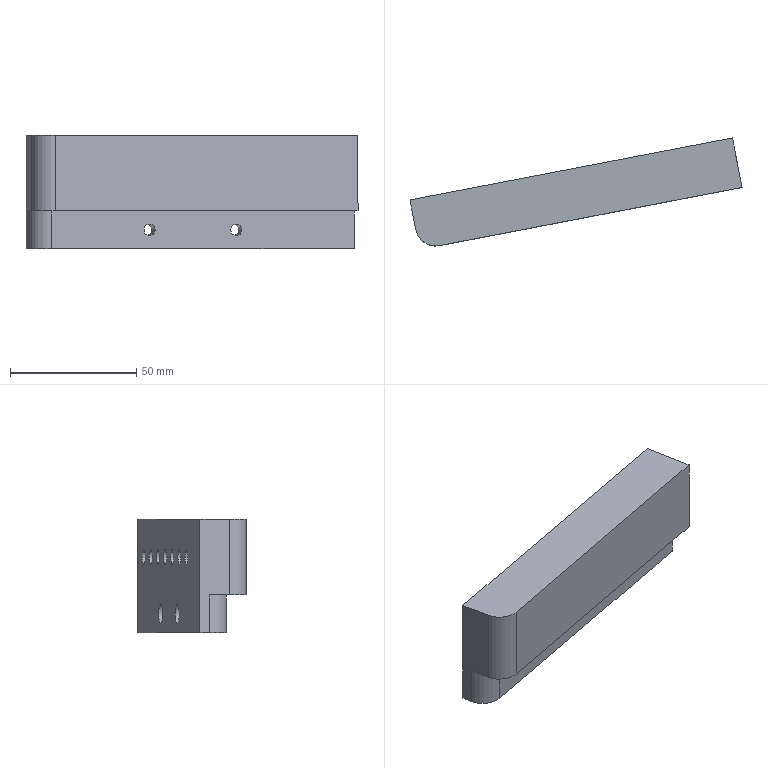Component | SolidWorks | SuctionCupMountingBlock2-1 | 1 solid | 37 faces | box 131.44 x 42.78 x 45 mm | volume 90210 mm3 | cylinder 26 | plane 11 | commonest cylinder face diameters 6 x14 8 x4 4.5 x4 10 x2 16 x2
build123d program:
from build123d import *

# Parameters (mm, degrees)
SKETCH2_W                                       = 20
SKETCH2_H                                       = 130
BOSS_EXTRUDE1_DEPTH                             = 30
SKETCH3_W                                       = 15
SKETCH3_H                                       = 130
BOSS_EXTRUDE2_DEPTH                             = 12
SKETCH4_R                                       = 3
CUT_EXTRUDE1_DEPTH                              = 11
SKETCH5_R                                       = 5
CUT_EXTRUDE2_DEPTH                              = 110
M4_HEX_SOCKET_HEAD_CAP_SCREW_CBORE1_D           = 4.5
M4_HEX_SOCKET_HEAD_CAP_SCREW_CBORE1_DEPTH       = 20
M4_HEX_SOCKET_HEAD_CAP_SCREW_CBORE1_CBORE_D     = 8
M4_HEX_SOCKET_HEAD_CAP_SCREW_CBORE1_CBORE_DEPTH = 4.6
M4_HEX_SOCKET_HEAD_CAP_SCREW_CBORE1_TIP         = 1.352
FILLET1_R                                       = 8


with BuildPart() as part:
    # Sketch2 → Boss-Extrude1 (new body)
    with BuildSketch(Plane.XY):
        with Locations((10, 65)):
            Rectangle(SKETCH2_W, SKETCH2_H)
    extrude(amount=BOSS_EXTRUDE1_DEPTH)

    # Sketch3 → Boss-Extrude2 (add)
    with BuildSketch(Plane(origin=(20, 0, 0), x_dir=(0, 0, -1), z_dir=(1, 0, 0))):
        with Locations((-37.5, 65)):
            Rectangle(SKETCH3_W, SKETCH3_H)
    extrude(amount=-BOSS_EXTRUDE2_DEPTH)

    # Sketch4 → Cut-Extrude1 (cut)
    with BuildSketch(Plane(origin=(20, 0, 0), x_dir=(0, 0, -1), z_dir=(1, 0, 0))):
        with Locations((-15, 118)):
            Circle(SKETCH4_R)
        with Locations((-15, 103)):
            Circle(SKETCH4_R)
        with Locations((-15, 88)):
            Circle(SKETCH4_R)
        with Locations((-15, 73)):
            Circle(SKETCH4_R)
        with Locations((-15, 58)):
            Circle(SKETCH4_R)
        with Locations((-15, 43)):
            Circle(SKETCH4_R)
        with Locations((-15, 28)):
            Circle(SKETCH4_R)
    extrude(amount=-CUT_EXTRUDE1_DEPTH, mode=Mode.SUBTRACT)

    # Sketch5 → Cut-Extrude2 (cut)
    with BuildSketch(Plane(origin=(0, 130, 0), x_dir=(1, 0, 0), z_dir=(0, 1, 0))):
        with Locations(Location((9, -15, 0), (0, 0, 270))):
            Circle(SKETCH5_R)
    extrude(amount=-CUT_EXTRUDE2_DEPTH, mode=Mode.SUBTRACT)

    # M4 Hex Socket Head Cap Screw CBORE1
    with Locations(Plane(origin=(20, 0, 0), x_dir=(0, 0, -1), z_dir=(1, 0, 0))):
        with Locations((-37.5, 82.5), (-37.5, 47.5)):
            CounterBoreHole(M4_HEX_SOCKET_HEAD_CAP_SCREW_CBORE1_D / 2, M4_HEX_SOCKET_HEAD_CAP_SCREW_CBORE1_CBORE_D / 2, M4_HEX_SOCKET_HEAD_CAP_SCREW_CBORE1_CBORE_DEPTH, depth=M4_HEX_SOCKET_HEAD_CAP_SCREW_CBORE1_DEPTH)
            with Locations((0, 0, -(M4_HEX_SOCKET_HEAD_CAP_SCREW_CBORE1_DEPTH + M4_HEX_SOCKET_HEAD_CAP_SCREW_CBORE1_TIP / 2))):  # 118° drill point
                Cone(0, M4_HEX_SOCKET_HEAD_CAP_SCREW_CBORE1_D / 2, M4_HEX_SOCKET_HEAD_CAP_SCREW_CBORE1_TIP, mode=Mode.SUBTRACT)

    # Fillet1
    fillet1_edges = [part.edges().sort_by_distance(p)[0] for p in [
        (0, 0, 15),
        (8, 0, 37.5),
    ]]
    fillet(fillet1_edges, radius=FILLET1_R)


solid = part.part

# Placed as in the assembly
solid = solid.moved(Location((-420.887, 84.424, 388.468), (-180, 0, -100.867)))